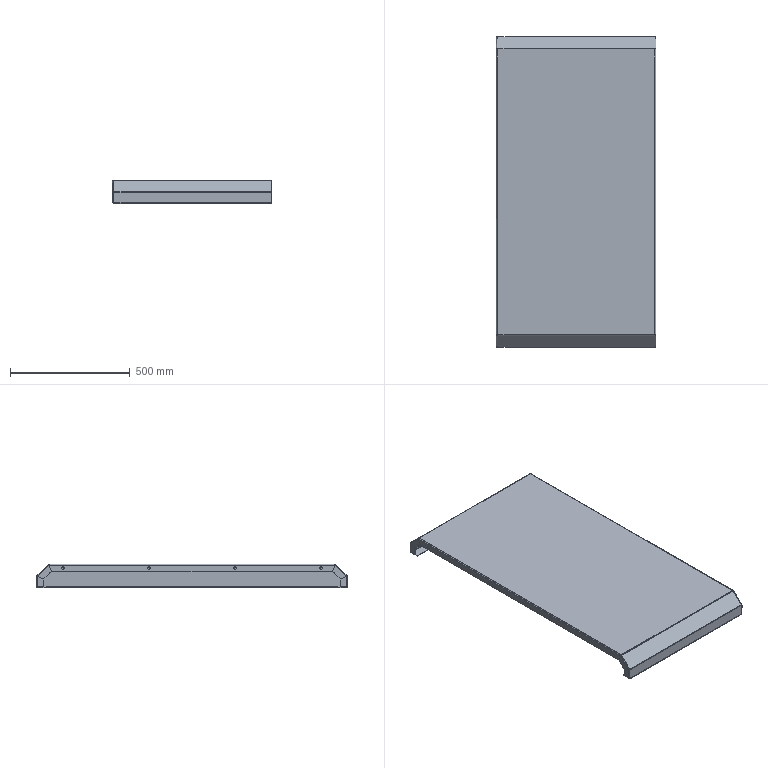Component | SolidWorks | RearTopCoverAssembly-1_RearTopCover-1 | 1 solid | 180 faces | volume 2412034 mm3 | plane 120 | cylinder 52 | spline 8 | commonest cylinder face diameters 10 x24 4 x15 8 x13 | material Plain Carbon Steel